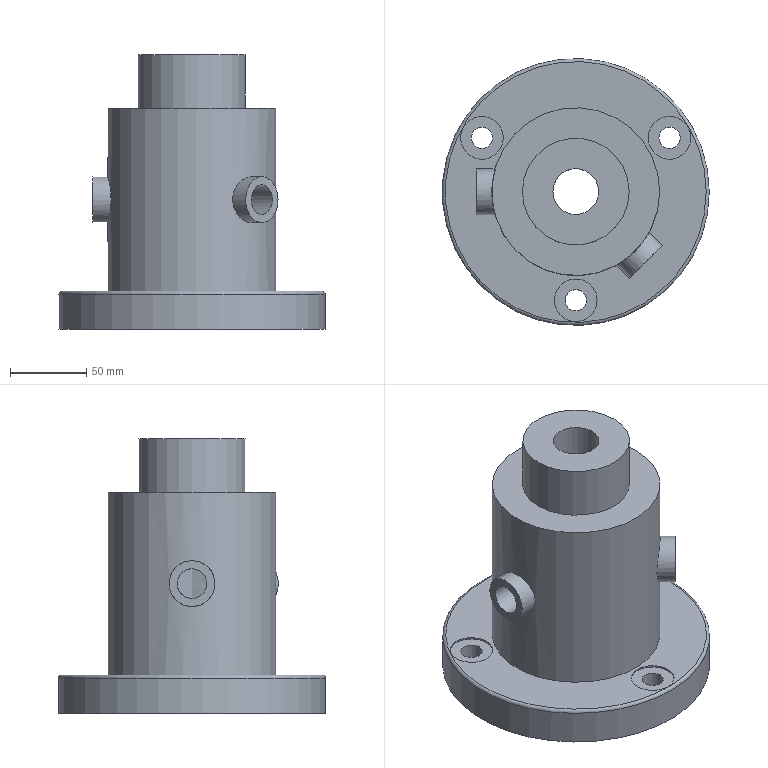Component | NX | VALVE_SEAT | 1 solid | 28 faces | volume 1539214 mm3 | cylinder 15 | plane 11 | cone 1 | torus 1 | commonest cylinder face diameters 14 x3 28 x3 30 x3 19.5 x2 110 x1 175 x1 70 x1 60 x1